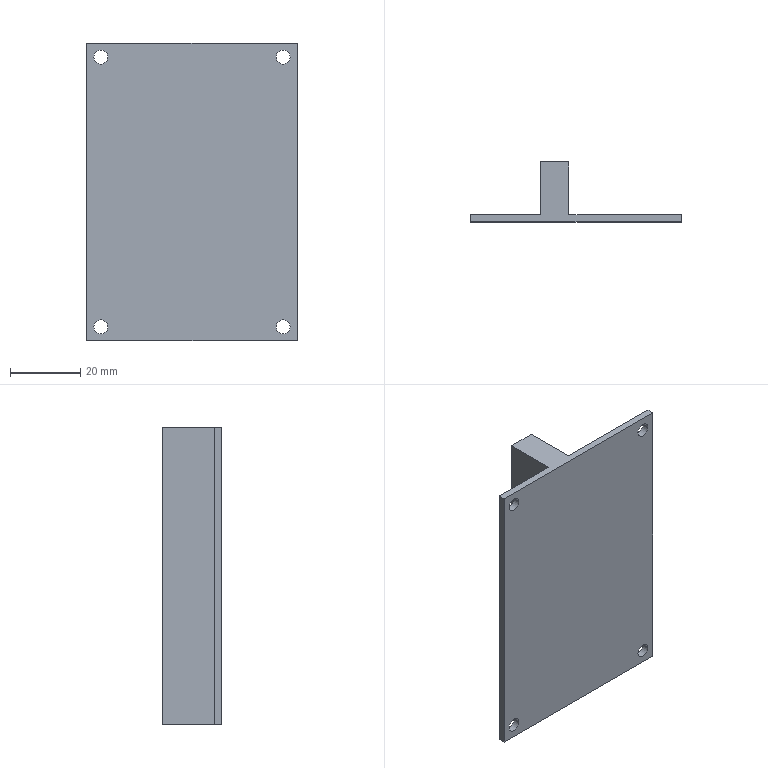Component | SolidWorks | WheelAssembly-1_CoverPlate-1 | 1 solid | 18 faces | box 60 x 17 x 85 mm | volume 20299 mm3 | plane 10 | cylinder 8 | commonest cylinder face diameters 4 x8
build123d program:
from build123d import *

# Parameters (mm, degrees)
SKETCH1_2_W          = 85
SKETCH1_2_H          = 60
BOSS_EXTRUDE1_DEPTH  = 2
SKETCH2_R            = 2
CUT_EXTRUDE1_2_DEPTH = 2
SKETCH3_W            = 8
SKETCH3_H            = 15.002
BOSS_EXTRUDE2_DEPTH  = 85


with BuildPart() as part:
    # Sketch1_2 → Boss-Extrude1 (new body)
    with BuildSketch(Plane(origin=(0, 0, 0), x_dir=(1, 0, 0), z_dir=(0, 1, 0))):
        Rectangle(SKETCH1_2_W, SKETCH1_2_H)
    extrude(amount=BOSS_EXTRUDE1_DEPTH)

    # Sketch2 → Cut-Extrude1_2 (cut)
    with BuildSketch(Plane(origin=(0, 2, 0), x_dir=(1, 0, 0), z_dir=(0, 1, 0))):
        with Locations(Location((-38.5, 26, 0), (0, 0, 270))):
            Circle(SKETCH2_R)
        with Locations(Location((38.5, 26, 0), (0, 0, 90))):
            Circle(SKETCH2_R)
        with Locations(Location((38.5, -26, 0), (0, 0, 270))):
            Circle(SKETCH2_R)
        with Locations(Location((-38.5, -26, 0), (0, 0, 90))):
            Circle(SKETCH2_R)
    extrude(amount=-CUT_EXTRUDE1_2_DEPTH, mode=Mode.SUBTRACT)

    # Sketch3 → Boss-Extrude2 (add)
    with BuildSketch(Plane.ZY.offset(42.5)):
        with Locations((-6, -7.499)):
            Rectangle(SKETCH3_W, SKETCH3_H)
    extrude(amount=-BOSS_EXTRUDE2_DEPTH)


solid = part.part

# Placed as in the assembly
solid = solid.moved(Location((-350, -148, -542.97), (180, 90, 0)))
STEP:
#1=COLOUR_RGB('',0.7922,0.8196,0.9333);
#2=FILL_AREA_STYLE_COLOUR('',#1);
#3=FILL_AREA_STYLE('',(#2));
#4=SURFACE_STYLE_FILL_AREA(#3);
#5=SURFACE_SIDE_STYLE('',(#4));
#6=SURFACE_STYLE_USAGE(.BOTH.,#5);
#7=PRESENTATION_STYLE_ASSIGNMENT((#6));
#8=CARTESIAN_POINT('',(-12.835,-5.827,-22.893));
#9=VERTEX_POINT('',#8);
#10=CARTESIAN_POINT('',(-12.677,-5.827,-22.893));
#11=VERTEX_POINT('',#10);
#12=CARTESIAN_POINT('',(-12.756,-5.827,-22.893));
#13=DIRECTION('',(-0.,-1.,0.));
#14=DIRECTION('',(-1.,0.,0.));
#15=AXIS2_PLACEMENT_3D('',#12,#13,#14);
#16=CIRCLE('',#15,0.07874);
#17=EDGE_CURVE('',#9,#11,#16,.T.);
#18=ORIENTED_EDGE('',*,*,#17,.F.);
#19=CARTESIAN_POINT('',(-12.835,-5.906,-22.893));
#20=VERTEX_POINT('',#19);
#21=CARTESIAN_POINT('',(-12.835,-5.827,-22.893));
#22=DIRECTION('',(-0.,-1.,0.));
#23=VECTOR('',#22,39.37);
#24=LINE('',#21,#23);
#25=EDGE_CURVE('',#9,#20,#24,.T.);
#26=ORIENTED_EDGE('',*,*,#25,.T.);
#27=CARTESIAN_POINT('',(-12.677,-5.906,-22.893));
#28=VERTEX_POINT('',#27);
#29=CARTESIAN_POINT('',(-12.756,-5.906,-22.893));
#30=DIRECTION('',(-0.,-1.,0.));
#31=DIRECTION('',(-1.,0.,0.));
#32=AXIS2_PLACEMENT_3D('',#29,#30,#31);
#33=CIRCLE('',#32,0.07874);
#34=EDGE_CURVE('',#20,#28,#33,.T.);
#35=ORIENTED_EDGE('',*,*,#34,.T.);
#36=CARTESIAN_POINT('',(-12.677,-5.827,-22.893));
#37=DIRECTION('',(-0.,-1.,0.));
#38=VECTOR('',#37,39.37);
#39=LINE('',#36,#38);
#40=EDGE_CURVE('',#11,#28,#39,.T.);
#41=ORIENTED_EDGE('',*,*,#40,.F.);
#42=EDGE_LOOP('',(#18,#26,#35,#41));
#43=FACE_OUTER_BOUND('',#42,.T.);
#44=CARTESIAN_POINT('',(-12.756,-5.827,-22.893));
#45=DIRECTION('',(-0.,-1.,0.));
#46=DIRECTION('',(1.,0.,0.));
#47=AXIS2_PLACEMENT_3D('',#44,#45,#46);
#48=CYLINDRICAL_SURFACE('',#47,0.07874);
#49=ADVANCED_FACE('',(#43),#48,.F.);
#50=CARTESIAN_POINT('',(-12.835,-5.827,-19.861));
#51=VERTEX_POINT('',#50);
#52=CARTESIAN_POINT('',(-12.677,-5.827,-19.861));
#53=VERTEX_POINT('',#52);
#54=CARTESIAN_POINT('',(-12.756,-5.827,-19.861));
#55=DIRECTION('',(-0.,-1.,0.));
#56=DIRECTION('',(1.,0.,0.));
#57=AXIS2_PLACEMENT_3D('',#54,#55,#56);
#58=CIRCLE('',#57,0.07874);
#59=EDGE_CURVE('',#51,#53,#58,.T.);
#60=ORIENTED_EDGE('',*,*,#59,.F.);
#61=CARTESIAN_POINT('',(-12.835,-5.906,-19.861));
#62=VERTEX_POINT('',#61);
#63=CARTESIAN_POINT('',(-12.835,-5.827,-19.861));
#64=DIRECTION('',(-0.,-1.,0.));
#65=VECTOR('',#64,39.37);
#66=LINE('',#63,#65);
#67=EDGE_CURVE('',#51,#62,#66,.T.);
#68=ORIENTED_EDGE('',*,*,#67,.T.);
#69=CARTESIAN_POINT('',(-12.677,-5.906,-19.861));
#70=VERTEX_POINT('',#69);
#71=CARTESIAN_POINT('',(-12.756,-5.906,-19.861));
#72=DIRECTION('',(-0.,-1.,0.));
#73=DIRECTION('',(1.,0.,0.));
#74=AXIS2_PLACEMENT_3D('',#71,#72,#73);
#75=CIRCLE('',#74,0.07874);
#76=EDGE_CURVE('',#62,#70,#75,.T.);
#77=ORIENTED_EDGE('',*,*,#76,.T.);
#78=CARTESIAN_POINT('',(-12.677,-5.827,-19.861));
#79=DIRECTION('',(-0.,-1.,0.));
#80=VECTOR('',#79,39.37);
#81=LINE('',#78,#80);
#82=EDGE_CURVE('',#53,#70,#81,.T.);
#83=ORIENTED_EDGE('',*,*,#82,.F.);
#84=EDGE_LOOP('',(#60,#68,#77,#83));
#85=FACE_OUTER_BOUND('',#84,.T.);
#86=CARTESIAN_POINT('',(-12.756,-5.827,-19.861));
#87=DIRECTION('',(-0.,-1.,0.));
#88=DIRECTION('',(1.,0.,0.));
#89=AXIS2_PLACEMENT_3D('',#86,#87,#88);
#90=CYLINDRICAL_SURFACE('',#89,0.07874);
#91=ADVANCED_FACE('',(#85),#90,.F.);
#92=CARTESIAN_POINT('',(-14.882,-5.827,-19.861));
#93=VERTEX_POINT('',#92);
#94=CARTESIAN_POINT('',(-14.724,-5.827,-19.861));
#95=VERTEX_POINT('',#94);
#96=CARTESIAN_POINT('',(-14.803,-5.827,-19.861));
#97=DIRECTION('',(-0.,-1.,0.));
#98=DIRECTION('',(-1.,0.,0.));
#99=AXIS2_PLACEMENT_3D('',#96,#97,#98);
#100=CIRCLE('',#99,0.07874);
#101=EDGE_CURVE('',#93,#95,#100,.T.);
#102=ORIENTED_EDGE('',*,*,#101,.F.);
#103=CARTESIAN_POINT('',(-14.882,-5.906,-19.861));
#104=VERTEX_POINT('',#103);
#105=CARTESIAN_POINT('',(-14.882,-5.827,-19.861));
#106=DIRECTION('',(-0.,-1.,0.));
#107=VECTOR('',#106,39.37);
#108=LINE('',#105,#107);
#109=EDGE_CURVE('',#93,#104,#108,.T.);
#110=ORIENTED_EDGE('',*,*,#109,.T.);
#111=CARTESIAN_POINT('',(-14.724,-5.906,-19.861));
#112=VERTEX_POINT('',#111);
#113=CARTESIAN_POINT('',(-14.803,-5.906,-19.861));
#114=DIRECTION('',(-0.,-1.,0.));
#115=DIRECTION('',(-1.,0.,0.));
#116=AXIS2_PLACEMENT_3D('',#113,#114,#115);
#117=CIRCLE('',#116,0.07874);
#118=EDGE_CURVE('',#104,#112,#117,.T.);
#119=ORIENTED_EDGE('',*,*,#118,.T.);
#120=CARTESIAN_POINT('',(-14.724,-5.827,-19.861));
#121=DIRECTION('',(-0.,-1.,0.));
#122=VECTOR('',#121,39.37);
#123=LINE('',#120,#122);
#124=EDGE_CURVE('',#95,#112,#123,.T.);
#125=ORIENTED_EDGE('',*,*,#124,.F.);
#126=EDGE_LOOP('',(#102,#110,#119,#125));
#127=FACE_OUTER_BOUND('',#126,.T.);
#128=CARTESIAN_POINT('',(-14.803,-5.827,-19.861));
#129=DIRECTION('',(-0.,-1.,0.));
#130=DIRECTION('',(1.,0.,0.));
#131=AXIS2_PLACEMENT_3D('',#128,#129,#130);
#132=CYLINDRICAL_SURFACE('',#131,0.07874);
#133=ADVANCED_FACE('',(#127),#132,.F.);
#134=CARTESIAN_POINT('',(-14.882,-5.827,-22.893));
#135=VERTEX_POINT('',#134);
#136=CARTESIAN_POINT('',(-14.724,-5.827,-22.893));
#137=VERTEX_POINT('',#136);
#138=CARTESIAN_POINT('',(-14.803,-5.827,-22.893));
#139=DIRECTION('',(-0.,-1.,0.));
#140=DIRECTION('',(1.,0.,0.));
#141=AXIS2_PLACEMENT_3D('',#138,#139,#140);
#142=CIRCLE('',#141,0.07874);
#143=EDGE_CURVE('',#135,#137,#142,.T.);
#144=ORIENTED_EDGE('',*,*,#143,.F.);
#145=CARTESIAN_POINT('',(-14.882,-5.906,-22.893));
#146=VERTEX_POINT('',#145);
#147=CARTESIAN_POINT('',(-14.882,-5.827,-22.893));
#148=DIRECTION('',(-0.,-1.,0.));
#149=VECTOR('',#148,39.37);
#150=LINE('',#147,#149);
#151=EDGE_CURVE('',#135,#146,#150,.T.);
#152=ORIENTED_EDGE('',*,*,#151,.T.);
#153=CARTESIAN_POINT('',(-14.724,-5.906,-22.893));
#154=VERTEX_POINT('',#153);
#155=CARTESIAN_POINT('',(-14.803,-5.906,-22.893));
#156=DIRECTION('',(-0.,-1.,0.));
#157=DIRECTION('',(1.,0.,0.));
#158=AXIS2_PLACEMENT_3D('',#155,#156,#157);
#159=CIRCLE('',#158,0.07874);
#160=EDGE_CURVE('',#146,#154,#159,.T.);
#161=ORIENTED_EDGE('',*,*,#160,.T.);
#162=CARTESIAN_POINT('',(-14.724,-5.827,-22.893));
#163=DIRECTION('',(-0.,-1.,0.));
#164=VECTOR('',#163,39.37);
#165=LINE('',#162,#164);
#166=EDGE_CURVE('',#137,#154,#165,.T.);
#167=ORIENTED_EDGE('',*,*,#166,.F.);
#168=EDGE_LOOP('',(#144,#152,#161,#167));
#169=FACE_OUTER_BOUND('',#168,.T.);
#170=CARTESIAN_POINT('',(-14.803,-5.827,-22.893));
#171=DIRECTION('',(-0.,-1.,0.));
#172=DIRECTION('',(1.,0.,0.));
#173=AXIS2_PLACEMENT_3D('',#170,#171,#172);
#174=CYLINDRICAL_SURFACE('',#173,0.07874);
#175=ADVANCED_FACE('',(#169),#174,.F.);
#176=CARTESIAN_POINT('',(-14.803,-5.827,-22.893));
#177=DIRECTION('',(-0.,-1.,0.));
#178=DIRECTION('',(1.,0.,0.));
#179=AXIS2_PLACEMENT_3D('',#176,#177,#178);
#180=CIRCLE('',#179,0.07874);
#181=EDGE_CURVE('',#137,#135,#180,.T.);
#182=ORIENTED_EDGE('',*,*,#181,.T.);
#183=ORIENTED_EDGE('',*,*,#143,.T.);
#184=EDGE_LOOP('',(#182,#183));
#185=FACE_BOUND('',#184,.T.);
#186=CARTESIAN_POINT('',(-14.803,-5.827,-19.861));
#187=DIRECTION('',(-0.,-1.,0.));
#188=DIRECTION('',(-1.,0.,0.));
#189=AXIS2_PLACEMENT_3D('',#186,#187,#188);
#190=CIRCLE('',#189,0.07874);
#191=EDGE_CURVE('',#95,#93,#190,.T.);
#192=ORIENTED_EDGE('',*,*,#191,.T.);
#193=ORIENTED_EDGE('',*,*,#101,.T.);
#194=EDGE_LOOP('',(#192,#193));
#195=FACE_BOUND('',#194,.T.);
#196=CARTESIAN_POINT('',(-14.173,-5.827,-19.704));
#197=VERTEX_POINT('',#196);
#198=CARTESIAN_POINT('',(-14.961,-5.827,-19.704));
#199=VERTEX_POINT('',#198);
#200=CARTESIAN_POINT('',(-14.961,-5.827,-19.704));
#201=DIRECTION('',(-1.,0.,0.));
#202=VECTOR('',#201,39.37);
#203=LINE('',#200,#202);
#204=EDGE_CURVE('',#197,#199,#203,.T.);
#205=ORIENTED_EDGE('',*,*,#204,.F.);
#206=CARTESIAN_POINT('',(-14.173,-5.827,-23.05));
#207=VERTEX_POINT('',#206);
#208=CARTESIAN_POINT('',(-14.173,-5.827,-21.377));
#209=DIRECTION('',(-0.,-0.,-1.));
#210=VECTOR('',#209,39.37);
#211=LINE('',#208,#210);
#212=EDGE_CURVE('',#197,#207,#211,.T.);
#213=ORIENTED_EDGE('',*,*,#212,.T.);
#214=CARTESIAN_POINT('',(-14.961,-5.827,-23.05));
#215=VERTEX_POINT('',#214);
#216=CARTESIAN_POINT('',(-14.961,-5.827,-23.05));
#217=DIRECTION('',(1.,-0.,-0.));
#218=VECTOR('',#217,39.37);
#219=LINE('',#216,#218);
#220=EDGE_CURVE('',#215,#207,#219,.T.);
#221=ORIENTED_EDGE('',*,*,#220,.F.);
#222=CARTESIAN_POINT('',(-14.961,-5.827,-23.05));
#223=DIRECTION('',(-0.,-0.,-1.));
#224=VECTOR('',#223,39.37);
#225=LINE('',#222,#224);
#226=EDGE_CURVE('',#199,#215,#225,.T.);
#227=ORIENTED_EDGE('',*,*,#226,.F.);
#228=EDGE_LOOP('',(#205,#213,#221,#227));
#229=FACE_OUTER_BOUND('',#228,.T.);
#230=CARTESIAN_POINT('',(-13.78,-5.827,-21.377));
#231=DIRECTION('',(-0.,-1.,0.));
#232=DIRECTION('',(1.,-0.,-0.));
#233=AXIS2_PLACEMENT_3D('',#230,#231,#232);
#234=PLANE('',#233);
#235=ADVANCED_FACE('',(#185,#195,#229),#234,.F.);
#236=CARTESIAN_POINT('',(-14.173,-5.236,-19.704));
#237=VERTEX_POINT('',#236);
#238=CARTESIAN_POINT('',(-14.173,-5.236,-19.704));
#239=DIRECTION('',(-0.,-1.,0.));
#240=VECTOR('',#239,39.37);
#241=LINE('',#238,#240);
#242=EDGE_CURVE('',#237,#197,#241,.T.);
#243=ORIENTED_EDGE('',*,*,#242,.T.);
#244=ORIENTED_EDGE('',*,*,#204,.T.);
#245=CARTESIAN_POINT('',(-14.961,-5.906,-19.704));
#246=VERTEX_POINT('',#245);
#247=CARTESIAN_POINT('',(-14.961,-5.906,-19.704));
#248=DIRECTION('',(0.,1.,-0.));
#249=VECTOR('',#248,39.37);
#250=LINE('',#247,#249);
#251=EDGE_CURVE('',#246,#199,#250,.T.);
#252=ORIENTED_EDGE('',*,*,#251,.F.);
#253=CARTESIAN_POINT('',(-12.598,-5.906,-19.704));
#254=VERTEX_POINT('',#253);
#255=CARTESIAN_POINT('',(-14.961,-5.906,-19.704));
#256=DIRECTION('',(-1.,0.,0.));
#257=VECTOR('',#256,39.37);
#258=LINE('',#255,#257);
#259=EDGE_CURVE('',#254,#246,#258,.T.);
#260=ORIENTED_EDGE('',*,*,#259,.F.);
#261=CARTESIAN_POINT('',(-12.598,-5.827,-19.704));
#262=VERTEX_POINT('',#261);
#263=CARTESIAN_POINT('',(-12.598,-5.906,-19.704));
#264=DIRECTION('',(0.,1.,-0.));
#265=VECTOR('',#264,39.37);
#266=LINE('',#263,#265);
#267=EDGE_CURVE('',#254,#262,#266,.T.);
#268=ORIENTED_EDGE('',*,*,#267,.T.);
#269=CARTESIAN_POINT('',(-13.858,-5.827,-19.704));
#270=VERTEX_POINT('',#269);
#271=CARTESIAN_POINT('',(-14.961,-5.827,-19.704));
#272=DIRECTION('',(-1.,0.,0.));
#273=VECTOR('',#272,39.37);
#274=LINE('',#271,#273);
#275=EDGE_CURVE('',#262,#270,#274,.T.);
#276=ORIENTED_EDGE('',*,*,#275,.T.);
#277=CARTESIAN_POINT('',(-13.858,-5.236,-19.704));
#278=VERTEX_POINT('',#277);
#279=CARTESIAN_POINT('',(-13.858,-5.236,-19.704));
#280=DIRECTION('',(-0.,1.,-0.));
#281=VECTOR('',#280,39.37);
#282=LINE('',#279,#281);
#283=EDGE_CURVE('',#270,#278,#282,.T.);
#284=ORIENTED_EDGE('',*,*,#283,.T.);
#285=CARTESIAN_POINT('',(-14.173,-5.236,-19.704));
#286=DIRECTION('',(-1.,0.,0.));
#287=VECTOR('',#286,39.37);
#288=LINE('',#285,#287);
#289=EDGE_CURVE('',#278,#237,#288,.T.);
#290=ORIENTED_EDGE('',*,*,#289,.T.);
#291=EDGE_LOOP('',(#243,#244,#252,#260,#268,#276,#284,#290));
#292=FACE_OUTER_BOUND('',#291,.T.);
#293=CARTESIAN_POINT('',(-14.961,-5.906,-19.704));
#294=DIRECTION('',(-0.,-0.,-1.));
#295=DIRECTION('',(1.,-0.,-0.));
#296=AXIS2_PLACEMENT_3D('',#293,#294,#295);
#297=PLANE('',#296);
#298=ADVANCED_FACE('',(#292),#297,.F.);
#299=ORIENTED_EDGE('',*,*,#226,.T.);
#300=CARTESIAN_POINT('',(-14.961,-5.906,-23.05));
#301=VERTEX_POINT('',#300);
#302=CARTESIAN_POINT('',(-14.961,-5.906,-23.05));
#303=DIRECTION('',(0.,1.,-0.));
#304=VECTOR('',#303,39.37);
#305=LINE('',#302,#304);
#306=EDGE_CURVE('',#301,#215,#305,.T.);
#307=ORIENTED_EDGE('',*,*,#306,.F.);
#308=CARTESIAN_POINT('',(-14.961,-5.906,-23.05));
#309=DIRECTION('',(-0.,-0.,-1.));
#310=VECTOR('',#309,39.37);
#311=LINE('',#308,#310);
#312=EDGE_CURVE('',#246,#301,#311,.T.);
#313=ORIENTED_EDGE('',*,*,#312,.F.);
#314=ORIENTED_EDGE('',*,*,#251,.T.);
#315=EDGE_LOOP('',(#299,#307,#313,#314));
#316=FACE_OUTER_BOUND('',#315,.T.);
#317=CARTESIAN_POINT('',(-14.961,-5.906,-23.05));
#318=DIRECTION('',(1.,-0.,-0.));
#319=DIRECTION('',(0.,0.,1.));
#320=AXIS2_PLACEMENT_3D('',#317,#318,#319);
#321=PLANE('',#320);
#322=ADVANCED_FACE('',(#316),#321,.F.);
#323=ORIENTED_EDGE('',*,*,#220,.T.);
#324=CARTESIAN_POINT('',(-14.173,-5.236,-23.05));
#325=VERTEX_POINT('',#324);
#326=CARTESIAN_POINT('',(-14.173,-5.236,-23.05));
#327=DIRECTION('',(0.,1.,-0.));
#328=VECTOR('',#327,39.37);
#329=LINE('',#326,#328);
#330=EDGE_CURVE('',#207,#325,#329,.T.);
#331=ORIENTED_EDGE('',*,*,#330,.T.);
#332=CARTESIAN_POINT('',(-13.858,-5.236,-23.05));
#333=VERTEX_POINT('',#332);
#334=CARTESIAN_POINT('',(-14.173,-5.236,-23.05));
#335=DIRECTION('',(1.,-0.,-0.));
#336=VECTOR('',#335,39.37);
#337=LINE('',#334,#336);
#338=EDGE_CURVE('',#325,#333,#337,.T.);
#339=ORIENTED_EDGE('',*,*,#338,.T.);
#340=CARTESIAN_POINT('',(-13.858,-5.827,-23.05));
#341=VERTEX_POINT('',#340);
#342=CARTESIAN_POINT('',(-13.858,-5.236,-23.05));
#343=DIRECTION('',(0.,-1.,0.));
#344=VECTOR('',#343,39.37);
#345=LINE('',#342,#344);
#346=EDGE_CURVE('',#333,#341,#345,.T.);
#347=ORIENTED_EDGE('',*,*,#346,.T.);
#348=CARTESIAN_POINT('',(-12.598,-5.827,-23.05));
#349=VERTEX_POINT('',#348);
#350=CARTESIAN_POINT('',(-14.961,-5.827,-23.05));
#351=DIRECTION('',(1.,-0.,-0.));
#352=VECTOR('',#351,39.37);
#353=LINE('',#350,#352);
#354=EDGE_CURVE('',#341,#349,#353,.T.);
#355=ORIENTED_EDGE('',*,*,#354,.T.);
#356=CARTESIAN_POINT('',(-12.598,-5.906,-23.05));
#357=VERTEX_POINT('',#356);
#358=CARTESIAN_POINT('',(-12.598,-5.906,-23.05));
#359=DIRECTION('',(0.,1.,-0.));
#360=VECTOR('',#359,39.37);
#361=LINE('',#358,#360);
#362=EDGE_CURVE('',#357,#349,#361,.T.);
#363=ORIENTED_EDGE('',*,*,#362,.F.);
#364=CARTESIAN_POINT('',(-14.961,-5.906,-23.05));
#365=DIRECTION('',(1.,-0.,-0.));
#366=VECTOR('',#365,39.37);
#367=LINE('',#364,#366);
#368=EDGE_CURVE('',#301,#357,#367,.T.);
#369=ORIENTED_EDGE('',*,*,#368,.F.);
#370=ORIENTED_EDGE('',*,*,#306,.T.);
#371=EDGE_LOOP('',(#323,#331,#339,#347,#355,#363,#369,#370));
#372=FACE_OUTER_BOUND('',#371,.T.);
#373=CARTESIAN_POINT('',(-14.961,-5.906,-23.05));
#374=DIRECTION('',(0.,0.,1.));
#375=DIRECTION('',(-1.,0.,0.));
#376=AXIS2_PLACEMENT_3D('',#373,#374,#375);
#377=PLANE('',#376);
#378=ADVANCED_FACE('',(#372),#377,.F.);
#379=CARTESIAN_POINT('',(-12.598,-5.827,-23.05));
#380=DIRECTION('',(0.,0.,1.));
#381=VECTOR('',#380,39.37);
#382=LINE('',#379,#381);
#383=EDGE_CURVE('',#349,#262,#382,.T.);
#384=ORIENTED_EDGE('',*,*,#383,.T.);
#385=ORIENTED_EDGE('',*,*,#267,.F.);
#386=CARTESIAN_POINT('',(-12.598,-5.906,-23.05));
#387=DIRECTION('',(0.,0.,1.));
#388=VECTOR('',#387,39.37);
#389=LINE('',#386,#388);
#390=EDGE_CURVE('',#357,#254,#389,.T.);
#391=ORIENTED_EDGE('',*,*,#390,.F.);
#392=ORIENTED_EDGE('',*,*,#362,.T.);
#393=EDGE_LOOP('',(#384,#385,#391,#392));
#394=FACE_OUTER_BOUND('',#393,.T.);
#395=CARTESIAN_POINT('',(-12.598,-5.906,-23.05));
#396=DIRECTION('',(-1.,0.,0.));
#397=DIRECTION('',(-0.,-0.,-1.));
#398=AXIS2_PLACEMENT_3D('',#395,#396,#397);
#399=PLANE('',#398);
#400=ADVANCED_FACE('',(#394),#399,.F.);
#401=CARTESIAN_POINT('',(-12.756,-5.906,-22.893));
#402=DIRECTION('',(-0.,-1.,0.));
#403=DIRECTION('',(-1.,0.,0.));
#404=AXIS2_PLACEMENT_3D('',#401,#402,#403);
#405=CIRCLE('',#404,0.07874);
#406=EDGE_CURVE('',#28,#20,#405,.T.);
#407=ORIENTED_EDGE('',*,*,#406,.F.);
#408=ORIENTED_EDGE('',*,*,#34,.F.);
#409=EDGE_LOOP('',(#407,#408));
#410=FACE_BOUND('',#409,.T.);
#411=CARTESIAN_POINT('',(-12.756,-5.906,-19.861));
#412=DIRECTION('',(-0.,-1.,0.));
#413=DIRECTION('',(1.,0.,0.));
#414=AXIS2_PLACEMENT_3D('',#411,#412,#413);
#415=CIRCLE('',#414,0.07874);
#416=EDGE_CURVE('',#70,#62,#415,.T.);
#417=ORIENTED_EDGE('',*,*,#416,.F.);
#418=ORIENTED_EDGE('',*,*,#76,.F.);
#419=EDGE_LOOP('',(#417,#418));
#420=FACE_BOUND('',#419,.T.);
#421=CARTESIAN_POINT('',(-14.803,-5.906,-19.861));
#422=DIRECTION('',(-0.,-1.,0.));
#423=DIRECTION('',(-1.,0.,0.));
#424=AXIS2_PLACEMENT_3D('',#421,#422,#423);
#425=CIRCLE('',#424,0.07874);
#426=EDGE_CURVE('',#112,#104,#425,.T.);
#427=ORIENTED_EDGE('',*,*,#426,.F.);
#428=ORIENTED_EDGE('',*,*,#118,.F.);
#429=EDGE_LOOP('',(#427,#428));
#430=FACE_BOUND('',#429,.T.);
#431=CARTESIAN_POINT('',(-14.803,-5.906,-22.893));
#432=DIRECTION('',(-0.,-1.,0.));
#433=DIRECTION('',(1.,0.,0.));
#434=AXIS2_PLACEMENT_3D('',#431,#432,#433);
#435=CIRCLE('',#434,0.07874);
#436=EDGE_CURVE('',#154,#146,#435,.T.);
#437=ORIENTED_EDGE('',*,*,#436,.F.);
#438=ORIENTED_EDGE('',*,*,#160,.F.);
#439=EDGE_LOOP('',(#437,#438));
#440=FACE_BOUND('',#439,.T.);
#441=ORIENTED_EDGE('',*,*,#259,.T.);
#442=ORIENTED_EDGE('',*,*,#312,.T.);
#443=ORIENTED_EDGE('',*,*,#368,.T.);
#444=ORIENTED_EDGE('',*,*,#390,.T.);
#445=EDGE_LOOP('',(#441,#442,#443,#444));
#446=FACE_OUTER_BOUND('',#445,.T.);
#447=CARTESIAN_POINT('',(-13.78,-5.906,-21.377));
#448=DIRECTION('',(-0.,-1.,0.));
#449=DIRECTION('',(1.,-0.,-0.));
#450=AXIS2_PLACEMENT_3D('',#447,#448,#449);
#451=PLANE('',#450);
#452=ADVANCED_FACE('',(#410,#420,#430,#440,#446),#451,.T.);
#453=CARTESIAN_POINT('',(-12.756,-5.827,-22.893));
#454=DIRECTION('',(-0.,-1.,0.));
#455=DIRECTION('',(-1.,0.,0.));
#456=AXIS2_PLACEMENT_3D('',#453,#454,#455);
#457=CIRCLE('',#456,0.07874);
#458=EDGE_CURVE('',#11,#9,#457,.T.);
#459=ORIENTED_EDGE('',*,*,#458,.T.);
#460=ORIENTED_EDGE('',*,*,#17,.T.);
#461=EDGE_LOOP('',(#459,#460));
#462=FACE_BOUND('',#461,.T.);
#463=CARTESIAN_POINT('',(-12.756,-5.827,-19.861));
#464=DIRECTION('',(-0.,-1.,0.));
#465=DIRECTION('',(1.,0.,0.));
#466=AXIS2_PLACEMENT_3D('',#463,#464,#465);
#467=CIRCLE('',#466,0.07874);
#468=EDGE_CURVE('',#53,#51,#467,.T.);
#469=ORIENTED_EDGE('',*,*,#468,.T.);
#470=ORIENTED_EDGE('',*,*,#59,.T.);
#471=EDGE_LOOP('',(#469,#470));
#472=FACE_BOUND('',#471,.T.);
#473=ORIENTED_EDGE('',*,*,#354,.F.);
#474=CARTESIAN_POINT('',(-13.858,-5.827,-21.377));
#475=DIRECTION('',(0.,0.,1.));
#476=VECTOR('',#475,39.37);
#477=LINE('',#474,#476);
#478=EDGE_CURVE('',#341,#270,#477,.T.);
#479=ORIENTED_EDGE('',*,*,#478,.T.);
#480=ORIENTED_EDGE('',*,*,#275,.F.);
#481=ORIENTED_EDGE('',*,*,#383,.F.);
#482=EDGE_LOOP('',(#473,#479,#480,#481));
#483=FACE_OUTER_BOUND('',#482,.T.);
#484=CARTESIAN_POINT('',(-13.78,-5.827,-21.377));
#485=DIRECTION('',(-0.,-1.,0.));
#486=DIRECTION('',(1.,-0.,-0.));
#487=AXIS2_PLACEMENT_3D('',#484,#485,#486);
#488=PLANE('',#487);
#489=ADVANCED_FACE('',(#462,#472,#483),#488,.F.);
#490=ORIENTED_EDGE('',*,*,#151,.F.);
#491=ORIENTED_EDGE('',*,*,#181,.F.);
#492=ORIENTED_EDGE('',*,*,#166,.T.);
#493=ORIENTED_EDGE('',*,*,#436,.T.);
#494=EDGE_LOOP('',(#490,#491,#492,#493));
#495=FACE_OUTER_BOUND('',#494,.T.);
#496=CARTESIAN_POINT('',(-14.803,-5.827,-22.893));
#497=DIRECTION('',(-0.,-1.,0.));
#498=DIRECTION('',(1.,0.,0.));
#499=AXIS2_PLACEMENT_3D('',#496,#497,#498);
#500=CYLINDRICAL_SURFACE('',#499,0.07874);
#501=ADVANCED_FACE('',(#495),#500,.F.);
#502=ORIENTED_EDGE('',*,*,#109,.F.);
#503=ORIENTED_EDGE('',*,*,#191,.F.);
#504=ORIENTED_EDGE('',*,*,#124,.T.);
#505=ORIENTED_EDGE('',*,*,#426,.T.);
#506=EDGE_LOOP('',(#502,#503,#504,#505));
#507=FACE_OUTER_BOUND('',#506,.T.);
#508=CARTESIAN_POINT('',(-14.803,-5.827,-19.861));
#509=DIRECTION('',(-0.,-1.,0.));
#510=DIRECTION('',(1.,0.,0.));
#511=AXIS2_PLACEMENT_3D('',#508,#509,#510);
#512=CYLINDRICAL_SURFACE('',#511,0.07874);
#513=ADVANCED_FACE('',(#507),#512,.F.);
#514=ORIENTED_EDGE('',*,*,#67,.F.);
#515=ORIENTED_EDGE('',*,*,#468,.F.);
#516=ORIENTED_EDGE('',*,*,#82,.T.);
#517=ORIENTED_EDGE('',*,*,#416,.T.);
#518=EDGE_LOOP('',(#514,#515,#516,#517));
#519=FACE_OUTER_BOUND('',#518,.T.);
#520=CARTESIAN_POINT('',(-12.756,-5.827,-19.861));
#521=DIRECTION('',(-0.,-1.,0.));
#522=DIRECTION('',(1.,0.,0.));
#523=AXIS2_PLACEMENT_3D('',#520,#521,#522);
#524=CYLINDRICAL_SURFACE('',#523,0.07874);
#525=ADVANCED_FACE('',(#519),#524,.F.);
#526=ORIENTED_EDGE('',*,*,#25,.F.);
#527=ORIENTED_EDGE('',*,*,#458,.F.);
#528=ORIENTED_EDGE('',*,*,#40,.T.);
#529=ORIENTED_EDGE('',*,*,#406,.T.);
#530=EDGE_LOOP('',(#526,#527,#528,#529));
#531=FACE_OUTER_BOUND('',#530,.T.);
#532=CARTESIAN_POINT('',(-12.756,-5.827,-22.893));
#533=DIRECTION('',(-0.,-1.,0.));
#534=DIRECTION('',(1.,0.,0.));
#535=AXIS2_PLACEMENT_3D('',#532,#533,#534);
#536=CYLINDRICAL_SURFACE('',#535,0.07874);
#537=ADVANCED_FACE('',(#531),#536,.F.);
#538=ORIENTED_EDGE('',*,*,#212,.F.);
#539=ORIENTED_EDGE('',*,*,#242,.F.);
#540=CARTESIAN_POINT('',(-14.173,-5.236,-19.034));
#541=DIRECTION('',(-0.,-0.,-1.));
#542=VECTOR('',#541,39.37);
#543=LINE('',#540,#542);
#544=EDGE_CURVE('',#237,#325,#543,.T.);
#545=ORIENTED_EDGE('',*,*,#544,.T.);
#546=ORIENTED_EDGE('',*,*,#330,.F.);
#547=EDGE_LOOP('',(#538,#539,#545,#546));
#548=FACE_OUTER_BOUND('',#547,.T.);
#549=CARTESIAN_POINT('',(-14.173,-5.236,-19.034));
#550=DIRECTION('',(-1.,0.,0.));
#551=DIRECTION('',(-0.,-0.,-1.));
#552=AXIS2_PLACEMENT_3D('',#549,#550,#551);
#553=PLANE('',#552);
#554=ADVANCED_FACE('',(#548),#553,.T.);
#555=ORIENTED_EDGE('',*,*,#478,.F.);
#556=ORIENTED_EDGE('',*,*,#346,.F.);
#557=CARTESIAN_POINT('',(-13.858,-5.236,-19.034));
#558=DIRECTION('',(-0.,-0.,-1.));
#559=VECTOR('',#558,39.37);
#560=LINE('',#557,#559);
#561=EDGE_CURVE('',#278,#333,#560,.T.);
#562=ORIENTED_EDGE('',*,*,#561,.F.);
#563=ORIENTED_EDGE('',*,*,#283,.F.);
#564=EDGE_LOOP('',(#555,#556,#562,#563));
#565=FACE_OUTER_BOUND('',#564,.T.);
#566=CARTESIAN_POINT('',(-13.858,-5.236,-19.034));
#567=DIRECTION('',(1.,0.,-0.));
#568=DIRECTION('',(-0.,1.,-0.));
#569=AXIS2_PLACEMENT_3D('',#566,#567,#568);
#570=PLANE('',#569);
#571=ADVANCED_FACE('',(#565),#570,.T.);
#572=ORIENTED_EDGE('',*,*,#289,.F.);
#573=ORIENTED_EDGE('',*,*,#561,.T.);
#574=ORIENTED_EDGE('',*,*,#338,.F.);
#575=ORIENTED_EDGE('',*,*,#544,.F.);
#576=EDGE_LOOP('',(#572,#573,#574,#575));
#577=FACE_OUTER_BOUND('',#576,.T.);
#578=CARTESIAN_POINT('',(-14.173,-5.236,-19.034));
#579=DIRECTION('',(0.,1.,-0.));
#580=DIRECTION('',(-1.,0.,0.));
#581=AXIS2_PLACEMENT_3D('',#578,#579,#580);
#582=PLANE('',#581);
#583=ADVANCED_FACE('',(#577),#582,.T.);
#584=CLOSED_SHELL('',(#49,#91,#133,#175,#235,#298,#322,#378,#400,#452,#489,#501,#513,#525,#537,#554,#571,#583));
#585=MANIFOLD_SOLID_BREP('',#584);
#586=STYLED_ITEM('',(#7),#585);
#587=(LENGTH_UNIT()NAMED_UNIT(*)SI_UNIT($,.METRE.));
#588=LENGTH_MEASURE_WITH_UNIT(LENGTH_MEASURE(0.0254),#587);
#589=DIMENSIONAL_EXPONENTS(1.,0.,0.,0.,0.,0.,0.);
#590=(CONVERSION_BASED_UNIT('',#588)LENGTH_UNIT()NAMED_UNIT(#589));
#591=UNCERTAINTY_MEASURE_WITH_UNIT(LENGTH_MEASURE(0.00001),#590,'','');
#592=(NAMED_UNIT(*)PLANE_ANGLE_UNIT()SI_UNIT($,.RADIAN.));
#593=(NAMED_UNIT(*)SI_UNIT($,.STERADIAN.)SOLID_ANGLE_UNIT());
#594=(GEOMETRIC_REPRESENTATION_CONTEXT(3)GLOBAL_UNCERTAINTY_ASSIGNED_CONTEXT((#591))GLOBAL_UNIT_ASSIGNED_CONTEXT((#590,#592,#593))REPRESENTATION_CONTEXT('',''));
#595=MECHANICAL_DESIGN_GEOMETRIC_PRESENTATION_REPRESENTATION('',(#586),#594);
#596=PRESENTATION_LAYER_ASSIGNMENT('','',(#586));
#597=CARTESIAN_POINT('',(0.,0.,0.));
#598=DIRECTION('',(0.,0.,1.));
#599=DIRECTION('',(1.,0.,0.));
#600=AXIS2_PLACEMENT_3D('',#597,#598,#599);
#601=(LENGTH_UNIT()NAMED_UNIT(*)SI_UNIT($,.METRE.));
#602=LENGTH_MEASURE_WITH_UNIT(LENGTH_MEASURE(0.0254),#601);
#603=DIMENSIONAL_EXPONENTS(1.,0.,0.,0.,0.,0.,0.);
#604=(CONVERSION_BASED_UNIT('',#602)LENGTH_UNIT()NAMED_UNIT(#603));
#605=UNCERTAINTY_MEASURE_WITH_UNIT(LENGTH_MEASURE(0.00001),#604,'','');
#606=(NAMED_UNIT(*)PLANE_ANGLE_UNIT()SI_UNIT($,.RADIAN.));
#607=(NAMED_UNIT(*)SI_UNIT($,.STERADIAN.)SOLID_ANGLE_UNIT());
#608=(GEOMETRIC_REPRESENTATION_CONTEXT(3)GLOBAL_UNCERTAINTY_ASSIGNED_CONTEXT((#605))GLOBAL_UNIT_ASSIGNED_CONTEXT((#604,#606,#607))REPRESENTATION_CONTEXT('',''));
#609=ADVANCED_BREP_SHAPE_REPRESENTATION('',(#585,#600),#608);